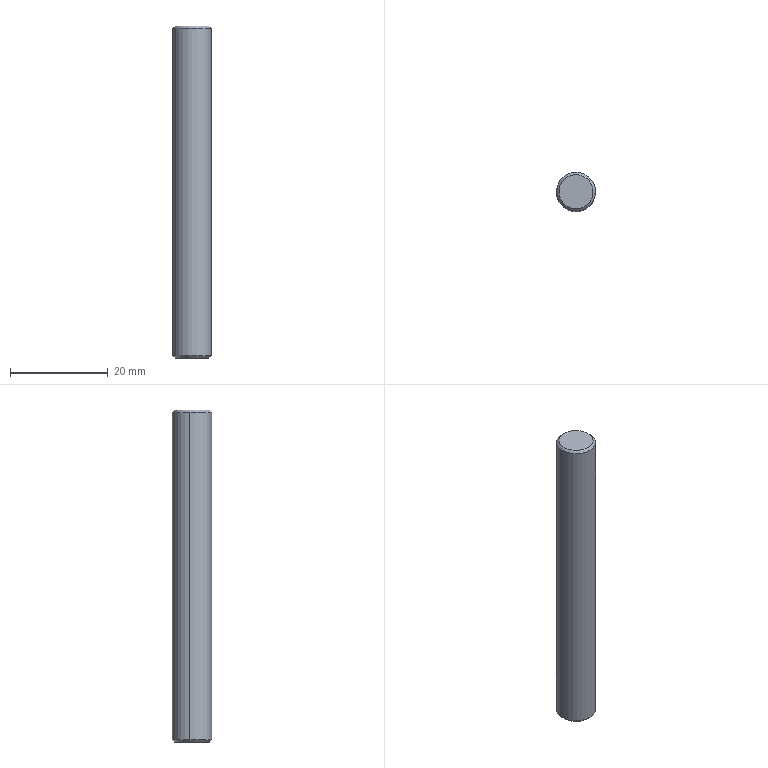Component | SolidWorks | JL001-05-02-1_JL001-05-01-005-1 | 1 solid | 8 faces | box 8 x 8 x 68 mm | volume 3412 mm3 | cone 4 | cylinder 2 | plane 2 | commonest cylinder face diameters 8 x2
build123d program:
from build123d import *

# Parameters (mm, degrees)
SKETCH1_R           = 4
BOSS_EXTRUDE1_DEPTH = 34
CHAMFER1_SIZE       = 0.5


with BuildPart() as part:
    # Sketch1 → Boss-Extrude1 (new, symmetric)
    with BuildSketch(Plane.XY):
        Circle(SKETCH1_R)
    extrude(amount=BOSS_EXTRUDE1_DEPTH, both=True)

    # Chamfer1
    chamfer1_edges = [part.edges().sort_by_distance(p)[0] for p in [
        (-4, 0, -34),
        (-4, 0, 34),
    ]]
    chamfer(chamfer1_edges, length=CHAMFER1_SIZE)


solid = part.part

# Placed as in the assembly
solid = solid.moved(Location((0, 1047.5, 63), (0, 0, 0)))
STEP:
#1=COLOUR_RGB('',0.7922,0.8196,0.9333);
#2=FILL_AREA_STYLE_COLOUR('',#1);
#3=FILL_AREA_STYLE('',(#2));
#4=SURFACE_STYLE_FILL_AREA(#3);
#5=SURFACE_SIDE_STYLE('',(#4));
#6=SURFACE_STYLE_USAGE(.BOTH.,#5);
#7=PRESENTATION_STYLE_ASSIGNMENT((#6));
#8=CARTESIAN_POINT('',(-0.137,41.255,3.819));
#9=VERTEX_POINT('',#8);
#10=CARTESIAN_POINT('',(0.137,41.225,3.819));
#11=VERTEX_POINT('',#10);
#12=CARTESIAN_POINT('',(-0.,41.24,3.819));
#13=DIRECTION('',(0.,0.,1.));
#14=DIRECTION('',(-0.9942,0.1077,0.));
#15=AXIS2_PLACEMENT_3D('',#12,#13,#14);
#16=CIRCLE('',#15,0.1378);
#17=EDGE_CURVE('',#9,#11,#16,.T.);
#18=ORIENTED_EDGE('',*,*,#17,.F.);
#19=CARTESIAN_POINT('',(-0.1566,41.257,3.799));
#20=VERTEX_POINT('',#19);
#21=CARTESIAN_POINT('',(-0.137,41.255,3.819));
#22=DIRECTION('',(-0.703,0.07615,-0.7071));
#23=VECTOR('',#22,39.37);
#24=LINE('',#21,#23);
#25=EDGE_CURVE('',#9,#20,#24,.T.);
#26=ORIENTED_EDGE('',*,*,#25,.T.);
#27=CARTESIAN_POINT('',(0.1566,41.223,3.799));
#28=VERTEX_POINT('',#27);
#29=CARTESIAN_POINT('',(-0.,41.24,3.799));
#30=DIRECTION('',(-0.,0.,-1.));
#31=DIRECTION('',(-0.9942,0.1077,0.));
#32=AXIS2_PLACEMENT_3D('',#29,#30,#31);
#33=CIRCLE('',#32,0.1575);
#34=EDGE_CURVE('',#28,#20,#33,.T.);
#35=ORIENTED_EDGE('',*,*,#34,.F.);
#36=CARTESIAN_POINT('',(0.137,41.225,3.819));
#37=DIRECTION('',(0.703,-0.07615,-0.7071));
#38=VECTOR('',#37,39.37);
#39=LINE('',#36,#38);
#40=EDGE_CURVE('',#11,#28,#39,.T.);
#41=ORIENTED_EDGE('',*,*,#40,.F.);
#42=EDGE_LOOP('',(#18,#26,#35,#41));
#43=FACE_OUTER_BOUND('',#42,.T.);
#44=CARTESIAN_POINT('',(-0.,41.24,3.819));
#45=DIRECTION('',(-0.,0.,-1.));
#46=DIRECTION('',(0.9942,-0.1077,0.));
#47=AXIS2_PLACEMENT_3D('',#44,#45,#46);
#48=CONICAL_SURFACE('',#47,0.1378,0.7854);
#49=ADVANCED_FACE('',(#43),#48,.T.);
#50=CARTESIAN_POINT('',(0.137,41.225,1.142));
#51=VERTEX_POINT('',#50);
#52=CARTESIAN_POINT('',(-0.137,41.255,1.142));
#53=VERTEX_POINT('',#52);
#54=CARTESIAN_POINT('',(-0.,41.24,1.142));
#55=DIRECTION('',(-0.,0.,-1.));
#56=DIRECTION('',(-0.9942,0.1077,0.));
#57=AXIS2_PLACEMENT_3D('',#54,#55,#56);
#58=CIRCLE('',#57,0.1378);
#59=EDGE_CURVE('',#51,#53,#58,.T.);
#60=ORIENTED_EDGE('',*,*,#59,.F.);
#61=CARTESIAN_POINT('',(0.1566,41.223,1.161));
#62=VERTEX_POINT('',#61);
#63=CARTESIAN_POINT('',(0.1566,41.223,1.161));
#64=DIRECTION('',(0.703,-0.07615,0.7071));
#65=VECTOR('',#64,39.37);
#66=LINE('',#63,#65);
#67=EDGE_CURVE('',#51,#62,#66,.T.);
#68=ORIENTED_EDGE('',*,*,#67,.T.);
#69=CARTESIAN_POINT('',(-0.1566,41.257,1.161));
#70=VERTEX_POINT('',#69);
#71=CARTESIAN_POINT('',(-0.,41.24,1.161));
#72=DIRECTION('',(0.,0.,1.));
#73=DIRECTION('',(-0.9942,0.1077,0.));
#74=AXIS2_PLACEMENT_3D('',#71,#72,#73);
#75=CIRCLE('',#74,0.1575);
#76=EDGE_CURVE('',#70,#62,#75,.T.);
#77=ORIENTED_EDGE('',*,*,#76,.F.);
#78=CARTESIAN_POINT('',(-0.1566,41.257,1.161));
#79=DIRECTION('',(-0.703,0.07615,0.7071));
#80=VECTOR('',#79,39.37);
#81=LINE('',#78,#80);
#82=EDGE_CURVE('',#53,#70,#81,.T.);
#83=ORIENTED_EDGE('',*,*,#82,.F.);
#84=EDGE_LOOP('',(#60,#68,#77,#83));
#85=FACE_OUTER_BOUND('',#84,.T.);
#86=CARTESIAN_POINT('',(-0.,41.24,1.161));
#87=DIRECTION('',(0.,0.,1.));
#88=DIRECTION('',(-0.9942,0.1077,0.));
#89=AXIS2_PLACEMENT_3D('',#86,#87,#88);
#90=CONICAL_SURFACE('',#89,0.1575,0.7854);
#91=ADVANCED_FACE('',(#85),#90,.T.);
#92=ORIENTED_EDGE('',*,*,#34,.T.);
#93=CARTESIAN_POINT('',(-0.1566,41.257,3.819));
#94=DIRECTION('',(-0.,0.,-1.));
#95=VECTOR('',#94,39.37);
#96=LINE('',#93,#95);
#97=EDGE_CURVE('',#20,#70,#96,.T.);
#98=ORIENTED_EDGE('',*,*,#97,.T.);
#99=ORIENTED_EDGE('',*,*,#76,.T.);
#100=CARTESIAN_POINT('',(0.1566,41.223,3.819));
#101=DIRECTION('',(-0.,0.,-1.));
#102=VECTOR('',#101,39.37);
#103=LINE('',#100,#102);
#104=EDGE_CURVE('',#28,#62,#103,.T.);
#105=ORIENTED_EDGE('',*,*,#104,.F.);
#106=EDGE_LOOP('',(#92,#98,#99,#105));
#107=FACE_OUTER_BOUND('',#106,.T.);
#108=CARTESIAN_POINT('',(-0.,41.24,3.819));
#109=DIRECTION('',(-0.,0.,-1.));
#110=DIRECTION('',(0.9942,-0.1077,0.));
#111=AXIS2_PLACEMENT_3D('',#108,#109,#110);
#112=CYLINDRICAL_SURFACE('',#111,0.1575);
#113=ADVANCED_FACE('',(#107),#112,.T.);
#114=ORIENTED_EDGE('',*,*,#97,.F.);
#115=CARTESIAN_POINT('',(-0.,41.24,3.799));
#116=DIRECTION('',(-0.,0.,-1.));
#117=DIRECTION('',(-0.9942,0.1077,0.));
#118=AXIS2_PLACEMENT_3D('',#115,#116,#117);
#119=CIRCLE('',#118,0.1575);
#120=EDGE_CURVE('',#20,#28,#119,.T.);
#121=ORIENTED_EDGE('',*,*,#120,.T.);
#122=ORIENTED_EDGE('',*,*,#104,.T.);
#123=CARTESIAN_POINT('',(-0.,41.24,1.161));
#124=DIRECTION('',(0.,0.,1.));
#125=DIRECTION('',(-0.9942,0.1077,0.));
#126=AXIS2_PLACEMENT_3D('',#123,#124,#125);
#127=CIRCLE('',#126,0.1575);
#128=EDGE_CURVE('',#62,#70,#127,.T.);
#129=ORIENTED_EDGE('',*,*,#128,.T.);
#130=EDGE_LOOP('',(#114,#121,#122,#129));
#131=FACE_OUTER_BOUND('',#130,.T.);
#132=CARTESIAN_POINT('',(-0.,41.24,3.819));
#133=DIRECTION('',(-0.,0.,-1.));
#134=DIRECTION('',(0.9942,-0.1077,0.));
#135=AXIS2_PLACEMENT_3D('',#132,#133,#134);
#136=CYLINDRICAL_SURFACE('',#135,0.1575);
#137=ADVANCED_FACE('',(#131),#136,.T.);
#138=CARTESIAN_POINT('',(-0.,41.24,3.819));
#139=DIRECTION('',(0.,0.,1.));
#140=DIRECTION('',(-0.9942,0.1077,0.));
#141=AXIS2_PLACEMENT_3D('',#138,#139,#140);
#142=CIRCLE('',#141,0.1378);
#143=EDGE_CURVE('',#11,#9,#142,.T.);
#144=ORIENTED_EDGE('',*,*,#143,.T.);
#145=ORIENTED_EDGE('',*,*,#17,.T.);
#146=EDGE_LOOP('',(#144,#145));
#147=FACE_OUTER_BOUND('',#146,.T.);
#148=CARTESIAN_POINT('',(-0.,41.24,3.819));
#149=DIRECTION('',(0.,0.,1.));
#150=DIRECTION('',(-0.9942,0.1077,0.));
#151=AXIS2_PLACEMENT_3D('',#148,#149,#150);
#152=PLANE('',#151);
#153=ADVANCED_FACE('',(#147),#152,.T.);
#154=CARTESIAN_POINT('',(-0.,41.24,1.142));
#155=DIRECTION('',(-0.,0.,-1.));
#156=DIRECTION('',(-0.9942,0.1077,0.));
#157=AXIS2_PLACEMENT_3D('',#154,#155,#156);
#158=CIRCLE('',#157,0.1378);
#159=EDGE_CURVE('',#53,#51,#158,.T.);
#160=ORIENTED_EDGE('',*,*,#159,.T.);
#161=ORIENTED_EDGE('',*,*,#59,.T.);
#162=EDGE_LOOP('',(#160,#161));
#163=FACE_OUTER_BOUND('',#162,.T.);
#164=CARTESIAN_POINT('',(-0.,41.24,1.142));
#165=DIRECTION('',(0.,0.,1.));
#166=DIRECTION('',(-0.9942,0.1077,0.));
#167=AXIS2_PLACEMENT_3D('',#164,#165,#166);
#168=PLANE('',#167);
#169=ADVANCED_FACE('',(#163),#168,.F.);
#170=ORIENTED_EDGE('',*,*,#67,.F.);
#171=ORIENTED_EDGE('',*,*,#159,.F.);
#172=ORIENTED_EDGE('',*,*,#82,.T.);
#173=ORIENTED_EDGE('',*,*,#128,.F.);
#174=EDGE_LOOP('',(#170,#171,#172,#173));
#175=FACE_OUTER_BOUND('',#174,.T.);
#176=CARTESIAN_POINT('',(-0.,41.24,1.161));
#177=DIRECTION('',(0.,0.,1.));
#178=DIRECTION('',(-0.9942,0.1077,0.));
#179=AXIS2_PLACEMENT_3D('',#176,#177,#178);
#180=CONICAL_SURFACE('',#179,0.1575,0.7854);
#181=ADVANCED_FACE('',(#175),#180,.T.);
#182=ORIENTED_EDGE('',*,*,#25,.F.);
#183=ORIENTED_EDGE('',*,*,#143,.F.);
#184=ORIENTED_EDGE('',*,*,#40,.T.);
#185=ORIENTED_EDGE('',*,*,#120,.F.);
#186=EDGE_LOOP('',(#182,#183,#184,#185));
#187=FACE_OUTER_BOUND('',#186,.T.);
#188=CARTESIAN_POINT('',(-0.,41.24,3.819));
#189=DIRECTION('',(-0.,0.,-1.));
#190=DIRECTION('',(0.9942,-0.1077,0.));
#191=AXIS2_PLACEMENT_3D('',#188,#189,#190);
#192=CONICAL_SURFACE('',#191,0.1378,0.7854);
#193=ADVANCED_FACE('',(#187),#192,.T.);
#194=CLOSED_SHELL('',(#49,#91,#113,#137,#153,#169,#181,#193));
#195=MANIFOLD_SOLID_BREP('',#194);
#196=STYLED_ITEM('',(#7),#195);
#197=(LENGTH_UNIT()NAMED_UNIT(*)SI_UNIT($,.METRE.));
#198=LENGTH_MEASURE_WITH_UNIT(LENGTH_MEASURE(0.0254),#197);
#199=DIMENSIONAL_EXPONENTS(1.,0.,0.,0.,0.,0.,0.);
#200=(CONVERSION_BASED_UNIT('',#198)LENGTH_UNIT()NAMED_UNIT(#199));
#201=UNCERTAINTY_MEASURE_WITH_UNIT(LENGTH_MEASURE(0.00001),#200,'','');
#202=(NAMED_UNIT(*)PLANE_ANGLE_UNIT()SI_UNIT($,.RADIAN.));
#203=(NAMED_UNIT(*)SI_UNIT($,.STERADIAN.)SOLID_ANGLE_UNIT());
#204=(GEOMETRIC_REPRESENTATION_CONTEXT(3)GLOBAL_UNCERTAINTY_ASSIGNED_CONTEXT((#201))GLOBAL_UNIT_ASSIGNED_CONTEXT((#200,#202,#203))REPRESENTATION_CONTEXT('',''));
#205=MECHANICAL_DESIGN_GEOMETRIC_PRESENTATION_REPRESENTATION('',(#196),#204);
#206=CARTESIAN_POINT('',(0.,0.,0.));
#207=DIRECTION('',(0.,0.,1.));
#208=DIRECTION('',(1.,0.,0.));
#209=AXIS2_PLACEMENT_3D('',#206,#207,#208);
#210=(LENGTH_UNIT()NAMED_UNIT(*)SI_UNIT($,.METRE.));
#211=LENGTH_MEASURE_WITH_UNIT(LENGTH_MEASURE(0.0254),#210);
#212=DIMENSIONAL_EXPONENTS(1.,0.,0.,0.,0.,0.,0.);
#213=(CONVERSION_BASED_UNIT('',#211)LENGTH_UNIT()NAMED_UNIT(#212));
#214=UNCERTAINTY_MEASURE_WITH_UNIT(LENGTH_MEASURE(0.00001),#213,'','');
#215=(NAMED_UNIT(*)PLANE_ANGLE_UNIT()SI_UNIT($,.RADIAN.));
#216=(NAMED_UNIT(*)SI_UNIT($,.STERADIAN.)SOLID_ANGLE_UNIT());
#217=(GEOMETRIC_REPRESENTATION_CONTEXT(3)GLOBAL_UNCERTAINTY_ASSIGNED_CONTEXT((#214))GLOBAL_UNIT_ASSIGNED_CONTEXT((#213,#215,#216))REPRESENTATION_CONTEXT('',''));
#218=ADVANCED_BREP_SHAPE_REPRESENTATION('',(#195,#209),#217);
#219=PRESENTATION_LAYER_ASSIGNMENT('','',(#196));